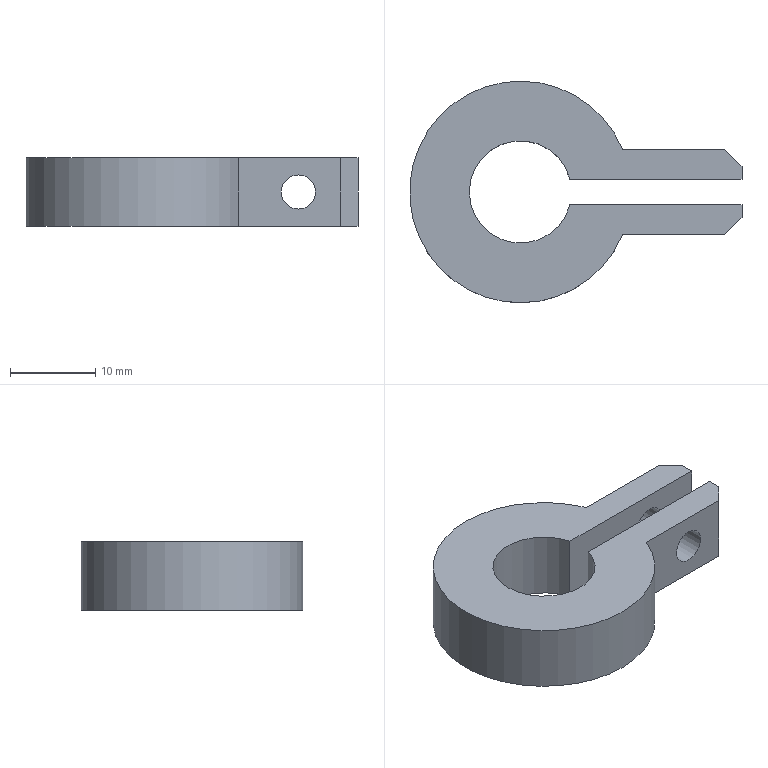Component | NX | RETAINING_RING | 1 solid | 14 faces | box 39 x 26 x 8 mm | volume 3807 mm3 | plane 10 | cylinder 4 | commonest cylinder face diameters 4.013 x2 26 x1 12 x1
STEP:
#1=CARTESIAN_POINT('',(0.,0.,0.));
#2=DIRECTION('',(0.,0.,1.));
#3=DIRECTION('',(1.,0.,0.));
#4=AXIS2_PLACEMENT_3D('',#1,#2,#3);
#5=CARTESIAN_POINT('',(33.5,3.,100.5));
#6=VERTEX_POINT('',#5);
#7=CARTESIAN_POINT('',(33.5,1.5,100.5));
#8=VERTEX_POINT('',#7);
#9=CARTESIAN_POINT('',(33.5,-0.,100.5));
#10=DIRECTION('',(0.,-1.,0.));
#11=VECTOR('',#10,1.);
#12=LINE('',#9,#11);
#13=CARTESIAN_POINT('',(33.5,-0.,108.5));
#14=DIRECTION('',(1.,0.,0.));
#15=DIRECTION('',(0.,0.,-1.));
#16=AXIS2_PLACEMENT_3D('',#13,#14,#15);
#17=PLANE('',#16);
#18=CARTESIAN_POINT('',(8.,0.));
#19=DIRECTION('',(0.,-1.));
#20=VECTOR('',#19,1.);
#21=LINE('',#18,#20);
#22=(GEOMETRIC_REPRESENTATION_CONTEXT(2)PARAMETRIC_REPRESENTATION_CONTEXT()REPRESENTATION_CONTEXT('',''));
#23=DEFINITIONAL_REPRESENTATION('',(#21),#22);
#24=PCURVE('',#17,#23);
#25=CARTESIAN_POINT('',(7.5,-0.,100.5));
#26=DIRECTION('',(0.,0.,-1.));
#27=DIRECTION('',(-1.,0.,0.));
#28=AXIS2_PLACEMENT_3D('',#25,#26,#27);
#29=PLANE('',#28);
#30=CARTESIAN_POINT('',(-26.,0.));
#31=DIRECTION('',(0.,-1.));
#32=VECTOR('',#31,1.);
#33=LINE('',#30,#32);
#34=(GEOMETRIC_REPRESENTATION_CONTEXT(2)PARAMETRIC_REPRESENTATION_CONTEXT()REPRESENTATION_CONTEXT('',''));
#35=DEFINITIONAL_REPRESENTATION('',(#33),#34);
#36=PCURVE('',#29,#35);
#37=SURFACE_CURVE('',#12,(#24,#36),.PCURVE_S1.);
#38=EDGE_CURVE('',#6,#8,#37,.T.);
#39=ORIENTED_EDGE('',*,*,#38,.F.);
#40=CARTESIAN_POINT('',(33.5,3.,108.5));
#41=VERTEX_POINT('',#40);
#42=CARTESIAN_POINT('',(33.5,3.,108.5));
#43=DIRECTION('',(0.,0.,1.));
#44=VECTOR('',#43,1.);
#45=LINE('',#42,#44);
#46=CARTESIAN_POINT('',(0.,3.));
#47=DIRECTION('',(-1.,0.));
#48=VECTOR('',#47,1.);
#49=LINE('',#46,#48);
#50=(GEOMETRIC_REPRESENTATION_CONTEXT(2)PARAMETRIC_REPRESENTATION_CONTEXT()REPRESENTATION_CONTEXT('',''));
#51=DEFINITIONAL_REPRESENTATION('',(#49),#50);
#52=PCURVE('',#17,#51);
#53=CARTESIAN_POINT('',(31.5,5.,108.5));
#54=DIRECTION('',(-0.7071,-0.7071,0.));
#55=DIRECTION('',(0.,0.,-1.));
#56=AXIS2_PLACEMENT_3D('',#53,#54,#55);
#57=PLANE('',#56);
#58=CARTESIAN_POINT('',(0.,2.828));
#59=DIRECTION('',(-1.,0.));
#60=VECTOR('',#59,1.);
#61=LINE('',#58,#60);
#62=(GEOMETRIC_REPRESENTATION_CONTEXT(2)PARAMETRIC_REPRESENTATION_CONTEXT()REPRESENTATION_CONTEXT('',''));
#63=DEFINITIONAL_REPRESENTATION('',(#61),#62);
#64=PCURVE('',#57,#63);
#65=SURFACE_CURVE('',#45,(#52,#64),.PCURVE_S1.);
#66=EDGE_CURVE('',#6,#41,#65,.T.);
#67=ORIENTED_EDGE('',*,*,#66,.T.);
#68=CARTESIAN_POINT('',(33.5,1.5,108.5));
#69=VERTEX_POINT('',#68);
#70=CARTESIAN_POINT('',(33.5,5.,108.5));
#71=DIRECTION('',(0.,-1.,0.));
#72=VECTOR('',#71,1.);
#73=LINE('',#70,#72);
#74=CARTESIAN_POINT('',(0.,5.));
#75=DIRECTION('',(0.,-1.));
#76=VECTOR('',#75,1.);
#77=LINE('',#74,#76);
#78=(GEOMETRIC_REPRESENTATION_CONTEXT(2)PARAMETRIC_REPRESENTATION_CONTEXT()REPRESENTATION_CONTEXT('',''));
#79=DEFINITIONAL_REPRESENTATION('',(#77),#78);
#80=PCURVE('',#17,#79);
#81=CARTESIAN_POINT('',(7.5,-0.,108.5));
#82=DIRECTION('',(0.,0.,-1.));
#83=DIRECTION('',(-1.,0.,0.));
#84=AXIS2_PLACEMENT_3D('',#81,#82,#83);
#85=PLANE('',#84);
#86=CARTESIAN_POINT('',(-26.,5.));
#87=DIRECTION('',(0.,-1.));
#88=VECTOR('',#87,1.);
#89=LINE('',#86,#88);
#90=(GEOMETRIC_REPRESENTATION_CONTEXT(2)PARAMETRIC_REPRESENTATION_CONTEXT()REPRESENTATION_CONTEXT('',''));
#91=DEFINITIONAL_REPRESENTATION('',(#89),#90);
#92=PCURVE('',#85,#91);
#93=SURFACE_CURVE('',#73,(#80,#92),.PCURVE_S1.);
#94=EDGE_CURVE('',#41,#69,#93,.T.);
#95=ORIENTED_EDGE('',*,*,#94,.T.);
#96=CARTESIAN_POINT('',(33.5,1.5,108.5));
#97=DIRECTION('',(0.,0.,1.));
#98=VECTOR('',#97,1.);
#99=LINE('',#96,#98);
#100=CARTESIAN_POINT('',(0.,1.5));
#101=DIRECTION('',(-1.,0.));
#102=VECTOR('',#101,1.);
#103=LINE('',#100,#102);
#104=(GEOMETRIC_REPRESENTATION_CONTEXT(2)PARAMETRIC_REPRESENTATION_CONTEXT()REPRESENTATION_CONTEXT('',''));
#105=DEFINITIONAL_REPRESENTATION('',(#103),#104);
#106=PCURVE('',#17,#105);
#107=CARTESIAN_POINT('',(36.5,1.5,95.5));
#108=DIRECTION('',(0.,1.,0.));
#109=DIRECTION('',(0.,0.,1.));
#110=AXIS2_PLACEMENT_3D('',#107,#108,#109);
#111=PLANE('',#110);
#112=CARTESIAN_POINT('',(13.,-3.));
#113=DIRECTION('',(1.,0.));
#114=VECTOR('',#113,1.);
#115=LINE('',#112,#114);
#116=(GEOMETRIC_REPRESENTATION_CONTEXT(2)PARAMETRIC_REPRESENTATION_CONTEXT()REPRESENTATION_CONTEXT('',''));
#117=DEFINITIONAL_REPRESENTATION('',(#115),#116);
#118=PCURVE('',#111,#117);
#119=SURFACE_CURVE('',#99,(#106,#118),.PCURVE_S1.);
#120=EDGE_CURVE('',#8,#69,#119,.T.);
#121=ORIENTED_EDGE('',*,*,#120,.F.);
#122=EDGE_LOOP('',(#39,#67,#95,#121));
#123=FACE_BOUND('',#122,.T.);
#124=ADVANCED_FACE('',(#123),#17,.T.);
#125=CARTESIAN_POINT('',(31.5,-5.,108.5));
#126=VERTEX_POINT('',#125);
#127=CARTESIAN_POINT('',(19.5,-5.,108.5));
#128=VERTEX_POINT('',#127);
#129=CARTESIAN_POINT('',(33.5,-5.,108.5));
#130=DIRECTION('',(-1.,0.,0.));
#131=VECTOR('',#130,1.);
#132=LINE('',#129,#131);
#133=CARTESIAN_POINT('',(-26.,-5.));
#134=DIRECTION('',(1.,0.));
#135=VECTOR('',#134,1.);
#136=LINE('',#133,#135);
#137=(GEOMETRIC_REPRESENTATION_CONTEXT(2)PARAMETRIC_REPRESENTATION_CONTEXT()REPRESENTATION_CONTEXT('',''));
#138=DEFINITIONAL_REPRESENTATION('',(#136),#137);
#139=PCURVE('',#85,#138);
#140=CARTESIAN_POINT('',(33.5,-5.,108.5));
#141=DIRECTION('',(0.,-1.,0.));
#142=DIRECTION('',(0.,0.,-1.));
#143=AXIS2_PLACEMENT_3D('',#140,#141,#142);
#144=PLANE('',#143);
#145=CARTESIAN_POINT('',(0.,0.));
#146=DIRECTION('',(0.,-1.));
#147=VECTOR('',#146,1.);
#148=LINE('',#145,#147);
#149=(GEOMETRIC_REPRESENTATION_CONTEXT(2)PARAMETRIC_REPRESENTATION_CONTEXT()REPRESENTATION_CONTEXT('',''));
#150=DEFINITIONAL_REPRESENTATION('',(#148),#149);
#151=PCURVE('',#144,#150);
#152=SURFACE_CURVE('',#132,(#139,#151),.PCURVE_S1.);
#153=EDGE_CURVE('',#126,#128,#152,.T.);
#154=ORIENTED_EDGE('',*,*,#153,.F.);
#155=CARTESIAN_POINT('',(33.5,-3.,108.5));
#156=VERTEX_POINT('',#155);
#157=CARTESIAN_POINT('',(33.5,-3.,108.5));
#158=DIRECTION('',(0.7071,0.7071,0.));
#159=VECTOR('',#158,1.);
#160=LINE('',#157,#159);
#161=CARTESIAN_POINT('',(-26.,-3.));
#162=DIRECTION('',(-0.7071,0.7071));
#163=VECTOR('',#162,1.);
#164=LINE('',#161,#163);
#165=(GEOMETRIC_REPRESENTATION_CONTEXT(2)PARAMETRIC_REPRESENTATION_CONTEXT()REPRESENTATION_CONTEXT('',''));
#166=DEFINITIONAL_REPRESENTATION('',(#164),#165);
#167=PCURVE('',#85,#166);
#168=CARTESIAN_POINT('',(33.5,-3.,108.5));
#169=DIRECTION('',(-0.7071,0.7071,0.));
#170=DIRECTION('',(0.,0.,-1.));
#171=AXIS2_PLACEMENT_3D('',#168,#169,#170);
#172=PLANE('',#171);
#173=CARTESIAN_POINT('',(0.,0.));
#174=DIRECTION('',(0.,-1.));
#175=VECTOR('',#174,1.);
#176=LINE('',#173,#175);
#177=(GEOMETRIC_REPRESENTATION_CONTEXT(2)PARAMETRIC_REPRESENTATION_CONTEXT()REPRESENTATION_CONTEXT('',''));
#178=DEFINITIONAL_REPRESENTATION('',(#176),#177);
#179=PCURVE('',#172,#178);
#180=SURFACE_CURVE('',#160,(#167,#179),.PCURVE_S1.);
#181=EDGE_CURVE('',#126,#156,#180,.T.);
#182=ORIENTED_EDGE('',*,*,#181,.T.);
#183=CARTESIAN_POINT('',(33.5,-1.5,108.5));
#184=VERTEX_POINT('',#183);
#185=CARTESIAN_POINT('',(33.5,5.,108.5));
#186=DIRECTION('',(0.,-1.,0.));
#187=VECTOR('',#186,1.);
#188=LINE('',#185,#187);
#189=CARTESIAN_POINT('',(-26.,5.));
#190=DIRECTION('',(0.,-1.));
#191=VECTOR('',#190,1.);
#192=LINE('',#189,#191);
#193=(GEOMETRIC_REPRESENTATION_CONTEXT(2)PARAMETRIC_REPRESENTATION_CONTEXT()REPRESENTATION_CONTEXT('',''));
#194=DEFINITIONAL_REPRESENTATION('',(#192),#193);
#195=PCURVE('',#85,#194);
#196=CARTESIAN_POINT('',(33.5,-0.,108.5));
#197=DIRECTION('',(1.,0.,0.));
#198=DIRECTION('',(0.,0.,-1.));
#199=AXIS2_PLACEMENT_3D('',#196,#197,#198);
#200=PLANE('',#199);
#201=CARTESIAN_POINT('',(0.,5.));
#202=DIRECTION('',(0.,-1.));
#203=VECTOR('',#202,1.);
#204=LINE('',#201,#203);
#205=(GEOMETRIC_REPRESENTATION_CONTEXT(2)PARAMETRIC_REPRESENTATION_CONTEXT()REPRESENTATION_CONTEXT('',''));
#206=DEFINITIONAL_REPRESENTATION('',(#204),#205);
#207=PCURVE('',#200,#206);
#208=SURFACE_CURVE('',#188,(#195,#207),.PCURVE_S1.);
#209=EDGE_CURVE('',#184,#156,#208,.T.);
#210=ORIENTED_EDGE('',*,*,#209,.F.);
#211=CARTESIAN_POINT('',(13.309,-1.5,108.5));
#212=VERTEX_POINT('',#211);
#213=CARTESIAN_POINT('',(12.,-1.5,108.5));
#214=DIRECTION('',(1.,0.,0.));
#215=VECTOR('',#214,1.);
#216=LINE('',#213,#215);
#217=CARTESIAN_POINT('',(-4.5,-1.5));
#218=DIRECTION('',(-1.,0.));
#219=VECTOR('',#218,1.);
#220=LINE('',#217,#219);
#221=(GEOMETRIC_REPRESENTATION_CONTEXT(2)PARAMETRIC_REPRESENTATION_CONTEXT()REPRESENTATION_CONTEXT('',''));
#222=DEFINITIONAL_REPRESENTATION('',(#220),#221);
#223=PCURVE('',#85,#222);
#224=CARTESIAN_POINT('',(12.,-1.5,95.5));
#225=DIRECTION('',(0.,-1.,0.));
#226=DIRECTION('',(0.,0.,-1.));
#227=AXIS2_PLACEMENT_3D('',#224,#225,#226);
#228=PLANE('',#227);
#229=CARTESIAN_POINT('',(-13.,0.));
#230=DIRECTION('',(0.,1.));
#231=VECTOR('',#230,1.);
#232=LINE('',#229,#231);
#233=(GEOMETRIC_REPRESENTATION_CONTEXT(2)PARAMETRIC_REPRESENTATION_CONTEXT()REPRESENTATION_CONTEXT('',''));
#234=DEFINITIONAL_REPRESENTATION('',(#232),#233);
#235=PCURVE('',#228,#234);
#236=SURFACE_CURVE('',#216,(#223,#235),.PCURVE_S1.);
#237=EDGE_CURVE('',#212,#184,#236,.T.);
#238=ORIENTED_EDGE('',*,*,#237,.F.);
#239=CARTESIAN_POINT('',(13.309,1.5,108.5));
#240=VERTEX_POINT('',#239);
#241=CARTESIAN_POINT('',(7.5,-0.,108.5));
#242=DIRECTION('',(0.,0.,-1.));
#243=DIRECTION('',(1.,0.,0.));
#244=AXIS2_PLACEMENT_3D('',#241,#242,#243);
#245=CIRCLE('',#244,6.);
#246=CARTESIAN_POINT('',(0.,0.));
#247=DIRECTION('',(-1.,0.));
#248=AXIS2_PLACEMENT_2D('',#246,#247);
#249=CIRCLE('',#248,6.);
#250=(GEOMETRIC_REPRESENTATION_CONTEXT(2)PARAMETRIC_REPRESENTATION_CONTEXT()REPRESENTATION_CONTEXT('',''));
#251=DEFINITIONAL_REPRESENTATION('',(#249),#250);
#252=PCURVE('',#85,#251);
#253=CARTESIAN_POINT('',(7.5,-0.,108.5));
#254=DIRECTION('',(0.,0.,-1.));
#255=DIRECTION('',(-1.,0.,0.));
#256=AXIS2_PLACEMENT_3D('',#253,#254,#255);
#257=CYLINDRICAL_SURFACE('',#256,6.);
#258=CARTESIAN_POINT('',(3.142,0.));
#259=DIRECTION('',(1.,0.));
#260=VECTOR('',#259,1.);
#261=LINE('',#258,#260);
#262=(GEOMETRIC_REPRESENTATION_CONTEXT(2)PARAMETRIC_REPRESENTATION_CONTEXT()REPRESENTATION_CONTEXT('',''));
#263=DEFINITIONAL_REPRESENTATION('',(#261),#262);
#264=PCURVE('',#257,#263);
#265=SURFACE_CURVE('',#245,(#252,#264),.PCURVE_S1.);
#266=EDGE_CURVE('',#212,#240,#265,.T.);
#267=ORIENTED_EDGE('',*,*,#266,.T.);
#268=CARTESIAN_POINT('',(36.5,1.5,108.5));
#269=DIRECTION('',(-1.,0.,0.));
#270=VECTOR('',#269,1.);
#271=LINE('',#268,#270);
#272=CARTESIAN_POINT('',(-29.,1.5));
#273=DIRECTION('',(1.,0.));
#274=VECTOR('',#273,1.);
#275=LINE('',#272,#274);
#276=(GEOMETRIC_REPRESENTATION_CONTEXT(2)PARAMETRIC_REPRESENTATION_CONTEXT()REPRESENTATION_CONTEXT('',''));
#277=DEFINITIONAL_REPRESENTATION('',(#275),#276);
#278=PCURVE('',#85,#277);
#279=CARTESIAN_POINT('',(13.,0.));
#280=DIRECTION('',(0.,-1.));
#281=VECTOR('',#280,1.);
#282=LINE('',#279,#281);
#283=(GEOMETRIC_REPRESENTATION_CONTEXT(2)PARAMETRIC_REPRESENTATION_CONTEXT()REPRESENTATION_CONTEXT('',''));
#284=DEFINITIONAL_REPRESENTATION('',(#282),#283);
#285=PCURVE('',#111,#284);
#286=SURFACE_CURVE('',#271,(#278,#285),.PCURVE_S1.);
#287=EDGE_CURVE('',#69,#240,#286,.T.);
#288=ORIENTED_EDGE('',*,*,#287,.F.);
#289=ORIENTED_EDGE('',*,*,#94,.F.);
#290=CARTESIAN_POINT('',(31.5,5.,108.5));
#291=VERTEX_POINT('',#290);
#292=CARTESIAN_POINT('',(31.5,5.,108.5));
#293=DIRECTION('',(-0.7071,0.7071,0.));
#294=VECTOR('',#293,1.);
#295=LINE('',#292,#294);
#296=CARTESIAN_POINT('',(-24.,5.));
#297=DIRECTION('',(0.7071,0.7071));
#298=VECTOR('',#297,1.);
#299=LINE('',#296,#298);
#300=(GEOMETRIC_REPRESENTATION_CONTEXT(2)PARAMETRIC_REPRESENTATION_CONTEXT()REPRESENTATION_CONTEXT('',''));
#301=DEFINITIONAL_REPRESENTATION('',(#299),#300);
#302=PCURVE('',#85,#301);
#303=CARTESIAN_POINT('',(0.,0.));
#304=DIRECTION('',(0.,-1.));
#305=VECTOR('',#304,1.);
#306=LINE('',#303,#305);
#307=(GEOMETRIC_REPRESENTATION_CONTEXT(2)PARAMETRIC_REPRESENTATION_CONTEXT()REPRESENTATION_CONTEXT('',''));
#308=DEFINITIONAL_REPRESENTATION('',(#306),#307);
#309=PCURVE('',#57,#308);
#310=SURFACE_CURVE('',#295,(#302,#309),.PCURVE_S1.);
#311=EDGE_CURVE('',#41,#291,#310,.T.);
#312=ORIENTED_EDGE('',*,*,#311,.T.);
#313=CARTESIAN_POINT('',(19.5,5.,108.5));
#314=VERTEX_POINT('',#313);
#315=CARTESIAN_POINT('',(19.5,5.,108.5));
#316=DIRECTION('',(1.,0.,0.));
#317=VECTOR('',#316,1.);
#318=LINE('',#315,#317);
#319=CARTESIAN_POINT('',(-12.,5.));
#320=DIRECTION('',(-1.,0.));
#321=VECTOR('',#320,1.);
#322=LINE('',#319,#321);
#323=(GEOMETRIC_REPRESENTATION_CONTEXT(2)PARAMETRIC_REPRESENTATION_CONTEXT()REPRESENTATION_CONTEXT('',''));
#324=DEFINITIONAL_REPRESENTATION('',(#322),#323);
#325=PCURVE('',#85,#324);
#326=CARTESIAN_POINT('',(19.5,5.,108.5));
#327=DIRECTION('',(0.,1.,0.));
#328=DIRECTION('',(0.,0.,1.));
#329=AXIS2_PLACEMENT_3D('',#326,#327,#328);
#330=PLANE('',#329);
#331=CARTESIAN_POINT('',(0.,0.));
#332=DIRECTION('',(0.,1.));
#333=VECTOR('',#332,1.);
#334=LINE('',#331,#333);
#335=(GEOMETRIC_REPRESENTATION_CONTEXT(2)PARAMETRIC_REPRESENTATION_CONTEXT()REPRESENTATION_CONTEXT('',''));
#336=DEFINITIONAL_REPRESENTATION('',(#334),#335);
#337=PCURVE('',#330,#336);
#338=SURFACE_CURVE('',#318,(#325,#337),.PCURVE_S1.);
#339=EDGE_CURVE('',#314,#291,#338,.T.);
#340=ORIENTED_EDGE('',*,*,#339,.F.);
#341=CARTESIAN_POINT('',(7.5,-0.,108.5));
#342=DIRECTION('',(0.,0.,-1.));
#343=DIRECTION('',(1.,0.,0.));
#344=AXIS2_PLACEMENT_3D('',#341,#342,#343);
#345=CIRCLE('',#344,13.);
#346=CARTESIAN_POINT('',(0.,0.));
#347=DIRECTION('',(-1.,0.));
#348=AXIS2_PLACEMENT_2D('',#346,#347);
#349=CIRCLE('',#348,13.);
#350=(GEOMETRIC_REPRESENTATION_CONTEXT(2)PARAMETRIC_REPRESENTATION_CONTEXT()REPRESENTATION_CONTEXT('',''));
#351=DEFINITIONAL_REPRESENTATION('',(#349),#350);
#352=PCURVE('',#85,#351);
#353=CARTESIAN_POINT('',(7.5,-0.,108.5));
#354=DIRECTION('',(0.,0.,-1.));
#355=DIRECTION('',(-1.,0.,0.));
#356=AXIS2_PLACEMENT_3D('',#353,#354,#355);
#357=CYLINDRICAL_SURFACE('',#356,13.);
#358=CARTESIAN_POINT('',(3.142,0.));
#359=DIRECTION('',(1.,0.));
#360=VECTOR('',#359,1.);
#361=LINE('',#358,#360);
#362=(GEOMETRIC_REPRESENTATION_CONTEXT(2)PARAMETRIC_REPRESENTATION_CONTEXT()REPRESENTATION_CONTEXT('',''));
#363=DEFINITIONAL_REPRESENTATION('',(#361),#362);
#364=PCURVE('',#357,#363);
#365=SURFACE_CURVE('',#345,(#352,#364),.PCURVE_S1.);
#366=EDGE_CURVE('',#128,#314,#365,.T.);
#367=ORIENTED_EDGE('',*,*,#366,.F.);
#368=EDGE_LOOP('',(#154,#182,#210,#238,#267,#288,#289,#312,#340,#367));
#369=FACE_BOUND('',#368,.T.);
#370=ADVANCED_FACE('',(#369),#85,.F.);
#371=CARTESIAN_POINT('',(19.5,-5.,100.5));
#372=VERTEX_POINT('',#371);
#373=CARTESIAN_POINT('',(19.5,5.,100.5));
#374=VERTEX_POINT('',#373);
#375=CARTESIAN_POINT('',(7.5,-0.,100.5));
#376=DIRECTION('',(0.,0.,-1.));
#377=DIRECTION('',(1.,0.,0.));
#378=AXIS2_PLACEMENT_3D('',#375,#376,#377);
#379=CIRCLE('',#378,13.);
#380=CARTESIAN_POINT('',(3.142,8.));
#381=DIRECTION('',(1.,0.));
#382=VECTOR('',#381,1.);
#383=LINE('',#380,#382);
#384=(GEOMETRIC_REPRESENTATION_CONTEXT(2)PARAMETRIC_REPRESENTATION_CONTEXT()REPRESENTATION_CONTEXT('',''));
#385=DEFINITIONAL_REPRESENTATION('',(#383),#384);
#386=PCURVE('',#357,#385);
#387=CARTESIAN_POINT('',(0.,0.));
#388=DIRECTION('',(-1.,0.));
#389=AXIS2_PLACEMENT_2D('',#387,#388);
#390=CIRCLE('',#389,13.);
#391=(GEOMETRIC_REPRESENTATION_CONTEXT(2)PARAMETRIC_REPRESENTATION_CONTEXT()REPRESENTATION_CONTEXT('',''));
#392=DEFINITIONAL_REPRESENTATION('',(#390),#391);
#393=PCURVE('',#29,#392);
#394=SURFACE_CURVE('',#379,(#386,#393),.PCURVE_S1.);
#395=EDGE_CURVE('',#372,#374,#394,.T.);
#396=ORIENTED_EDGE('',*,*,#395,.F.);
#397=CARTESIAN_POINT('',(19.5,-5.,108.5));
#398=DIRECTION('',(0.,0.,-1.));
#399=VECTOR('',#398,1.);
#400=LINE('',#397,#399);
#401=CARTESIAN_POINT('',(3.536,0.));
#402=DIRECTION('',(0.,1.));
#403=VECTOR('',#402,1.);
#404=LINE('',#401,#403);
#405=(GEOMETRIC_REPRESENTATION_CONTEXT(2)PARAMETRIC_REPRESENTATION_CONTEXT()REPRESENTATION_CONTEXT('',''));
#406=DEFINITIONAL_REPRESENTATION('',(#404),#405);
#407=PCURVE('',#357,#406);
#408=CARTESIAN_POINT('',(0.,-14.));
#409=DIRECTION('',(1.,0.));
#410=VECTOR('',#409,1.);
#411=LINE('',#408,#410);
#412=(GEOMETRIC_REPRESENTATION_CONTEXT(2)PARAMETRIC_REPRESENTATION_CONTEXT()REPRESENTATION_CONTEXT('',''));
#413=DEFINITIONAL_REPRESENTATION('',(#411),#412);
#414=PCURVE('',#144,#413);
#415=SURFACE_CURVE('',#400,(#407,#414),.PCURVE_S1.);
#416=EDGE_CURVE('',#128,#372,#415,.T.);
#417=ORIENTED_EDGE('',*,*,#416,.F.);
#418=ORIENTED_EDGE('',*,*,#366,.T.);
#419=CARTESIAN_POINT('',(19.5,5.,108.5));
#420=DIRECTION('',(0.,0.,-1.));
#421=VECTOR('',#420,1.);
#422=LINE('',#419,#421);
#423=CARTESIAN_POINT('',(9.03,0.));
#424=DIRECTION('',(0.,1.));
#425=VECTOR('',#424,1.);
#426=LINE('',#423,#425);
#427=(GEOMETRIC_REPRESENTATION_CONTEXT(2)PARAMETRIC_REPRESENTATION_CONTEXT()REPRESENTATION_CONTEXT('',''));
#428=DEFINITIONAL_REPRESENTATION('',(#426),#427);
#429=PCURVE('',#357,#428);
#430=CARTESIAN_POINT('',(0.,0.));
#431=DIRECTION('',(-1.,0.));
#432=VECTOR('',#431,1.);
#433=LINE('',#430,#432);
#434=(GEOMETRIC_REPRESENTATION_CONTEXT(2)PARAMETRIC_REPRESENTATION_CONTEXT()REPRESENTATION_CONTEXT('',''));
#435=DEFINITIONAL_REPRESENTATION('',(#433),#434);
#436=PCURVE('',#330,#435);
#437=SURFACE_CURVE('',#422,(#429,#436),.PCURVE_S1.);
#438=EDGE_CURVE('',#314,#374,#437,.T.);
#439=ORIENTED_EDGE('',*,*,#438,.T.);
#440=EDGE_LOOP('',(#396,#417,#418,#439));
#441=FACE_BOUND('',#440,.T.);
#442=ADVANCED_FACE('',(#441),#357,.T.);
#443=CARTESIAN_POINT('',(26.5,5.,106.507));
#444=VERTEX_POINT('',#443);
#445=CARTESIAN_POINT('',(26.5,5.,104.5));
#446=DIRECTION('',(0.,1.,0.));
#447=DIRECTION('',(0.,0.,1.));
#448=AXIS2_PLACEMENT_3D('',#445,#446,#447);
#449=CIRCLE('',#448,2.007);
#450=CARTESIAN_POINT('',(-4.,7.));
#451=DIRECTION('',(1.,0.));
#452=AXIS2_PLACEMENT_2D('',#450,#451);
#453=CIRCLE('',#452,2.007);
#454=(GEOMETRIC_REPRESENTATION_CONTEXT(2)PARAMETRIC_REPRESENTATION_CONTEXT()REPRESENTATION_CONTEXT('',''));
#455=DEFINITIONAL_REPRESENTATION('',(#453),#454);
#456=PCURVE('',#330,#455);
#457=CARTESIAN_POINT('',(26.5,-6.,104.5));
#458=DIRECTION('',(0.,1.,0.));
#459=DIRECTION('',(1.,0.,0.));
#460=AXIS2_PLACEMENT_3D('',#457,#458,#459);
#461=CYLINDRICAL_SURFACE('',#460,2.007);
#462=CARTESIAN_POINT('',(4.712,11.));
#463=DIRECTION('',(1.,0.));
#464=VECTOR('',#463,1.);
#465=LINE('',#462,#464);
#466=(GEOMETRIC_REPRESENTATION_CONTEXT(2)PARAMETRIC_REPRESENTATION_CONTEXT()REPRESENTATION_CONTEXT('',''));
#467=DEFINITIONAL_REPRESENTATION('',(#465),#466);
#468=PCURVE('',#461,#467);
#469=SURFACE_CURVE('',#449,(#456,#468),.PCURVE_S1.);
#470=EDGE_CURVE('',#444,#444,#469,.T.);
#471=ORIENTED_EDGE('',*,*,#470,.F.);
#472=EDGE_LOOP('',(#471));
#473=FACE_BOUND('',#472,.T.);
#474=ORIENTED_EDGE('',*,*,#339,.T.);
#475=CARTESIAN_POINT('',(31.5,5.,100.5));
#476=VERTEX_POINT('',#475);
#477=CARTESIAN_POINT('',(31.5,5.,108.5));
#478=DIRECTION('',(0.,0.,-1.));
#479=VECTOR('',#478,1.);
#480=LINE('',#477,#479);
#481=CARTESIAN_POINT('',(0.,12.));
#482=DIRECTION('',(-1.,0.));
#483=VECTOR('',#482,1.);
#484=LINE('',#481,#483);
#485=(GEOMETRIC_REPRESENTATION_CONTEXT(2)PARAMETRIC_REPRESENTATION_CONTEXT()REPRESENTATION_CONTEXT('',''));
#486=DEFINITIONAL_REPRESENTATION('',(#484),#485);
#487=PCURVE('',#330,#486);
#488=CARTESIAN_POINT('',(0.,0.));
#489=DIRECTION('',(1.,0.));
#490=VECTOR('',#489,1.);
#491=LINE('',#488,#490);
#492=(GEOMETRIC_REPRESENTATION_CONTEXT(2)PARAMETRIC_REPRESENTATION_CONTEXT()REPRESENTATION_CONTEXT('',''));
#493=DEFINITIONAL_REPRESENTATION('',(#491),#492);
#494=PCURVE('',#57,#493);
#495=SURFACE_CURVE('',#480,(#487,#494),.PCURVE_S1.);
#496=EDGE_CURVE('',#291,#476,#495,.T.);
#497=ORIENTED_EDGE('',*,*,#496,.T.);
#498=CARTESIAN_POINT('',(19.5,5.,100.5));
#499=DIRECTION('',(1.,0.,0.));
#500=VECTOR('',#499,1.);
#501=LINE('',#498,#500);
#502=CARTESIAN_POINT('',(-8.,0.));
#503=DIRECTION('',(0.,1.));
#504=VECTOR('',#503,1.);
#505=LINE('',#502,#504);
#506=(GEOMETRIC_REPRESENTATION_CONTEXT(2)PARAMETRIC_REPRESENTATION_CONTEXT()REPRESENTATION_CONTEXT('',''));
#507=DEFINITIONAL_REPRESENTATION('',(#505),#506);
#508=PCURVE('',#330,#507);
#509=CARTESIAN_POINT('',(-12.,5.));
#510=DIRECTION('',(-1.,0.));
#511=VECTOR('',#510,1.);
#512=LINE('',#509,#511);
#513=(GEOMETRIC_REPRESENTATION_CONTEXT(2)PARAMETRIC_REPRESENTATION_CONTEXT()REPRESENTATION_CONTEXT('',''));
#514=DEFINITIONAL_REPRESENTATION('',(#512),#513);
#515=PCURVE('',#29,#514);
#516=SURFACE_CURVE('',#501,(#508,#515),.PCURVE_S1.);
#517=EDGE_CURVE('',#374,#476,#516,.T.);
#518=ORIENTED_EDGE('',*,*,#517,.F.);
#519=ORIENTED_EDGE('',*,*,#438,.F.);
#520=EDGE_LOOP('',(#474,#497,#518,#519));
#521=FACE_BOUND('',#520,.T.);
#522=ADVANCED_FACE('',(#473,#521),#330,.T.);
#523=ORIENTED_EDGE('',*,*,#209,.T.);
#524=CARTESIAN_POINT('',(33.5,-3.,100.5));
#525=VERTEX_POINT('',#524);
#526=CARTESIAN_POINT('',(33.5,-3.,108.5));
#527=DIRECTION('',(0.,0.,-1.));
#528=VECTOR('',#527,1.);
#529=LINE('',#526,#528);
#530=CARTESIAN_POINT('',(0.,-3.));
#531=DIRECTION('',(1.,0.));
#532=VECTOR('',#531,1.);
#533=LINE('',#530,#532);
#534=(GEOMETRIC_REPRESENTATION_CONTEXT(2)PARAMETRIC_REPRESENTATION_CONTEXT()REPRESENTATION_CONTEXT('',''));
#535=DEFINITIONAL_REPRESENTATION('',(#533),#534);
#536=PCURVE('',#200,#535);
#537=CARTESIAN_POINT('',(0.,0.));
#538=DIRECTION('',(1.,0.));
#539=VECTOR('',#538,1.);
#540=LINE('',#537,#539);
#541=(GEOMETRIC_REPRESENTATION_CONTEXT(2)PARAMETRIC_REPRESENTATION_CONTEXT()REPRESENTATION_CONTEXT('',''));
#542=DEFINITIONAL_REPRESENTATION('',(#540),#541);
#543=PCURVE('',#172,#542);
#544=SURFACE_CURVE('',#529,(#536,#543),.PCURVE_S1.);
#545=EDGE_CURVE('',#156,#525,#544,.T.);
#546=ORIENTED_EDGE('',*,*,#545,.T.);
#547=CARTESIAN_POINT('',(33.5,-1.5,100.5));
#548=VERTEX_POINT('',#547);
#549=CARTESIAN_POINT('',(33.5,-0.,100.5));
#550=DIRECTION('',(0.,-1.,0.));
#551=VECTOR('',#550,1.);
#552=LINE('',#549,#551);
#553=CARTESIAN_POINT('',(8.,0.));
#554=DIRECTION('',(0.,-1.));
#555=VECTOR('',#554,1.);
#556=LINE('',#553,#555);
#557=(GEOMETRIC_REPRESENTATION_CONTEXT(2)PARAMETRIC_REPRESENTATION_CONTEXT()REPRESENTATION_CONTEXT('',''));
#558=DEFINITIONAL_REPRESENTATION('',(#556),#557);
#559=PCURVE('',#200,#558);
#560=CARTESIAN_POINT('',(-26.,0.));
#561=DIRECTION('',(0.,-1.));
#562=VECTOR('',#561,1.);
#563=LINE('',#560,#562);
#564=(GEOMETRIC_REPRESENTATION_CONTEXT(2)PARAMETRIC_REPRESENTATION_CONTEXT()REPRESENTATION_CONTEXT('',''));
#565=DEFINITIONAL_REPRESENTATION('',(#563),#564);
#566=PCURVE('',#29,#565);
#567=SURFACE_CURVE('',#552,(#559,#566),.PCURVE_S1.);
#568=EDGE_CURVE('',#548,#525,#567,.T.);
#569=ORIENTED_EDGE('',*,*,#568,.F.);
#570=CARTESIAN_POINT('',(33.5,-1.5,108.5));
#571=DIRECTION('',(0.,0.,-1.));
#572=VECTOR('',#571,1.);
#573=LINE('',#570,#572);
#574=CARTESIAN_POINT('',(0.,-1.5));
#575=DIRECTION('',(1.,0.));
#576=VECTOR('',#575,1.);
#577=LINE('',#574,#576);
#578=(GEOMETRIC_REPRESENTATION_CONTEXT(2)PARAMETRIC_REPRESENTATION_CONTEXT()REPRESENTATION_CONTEXT('',''));
#579=DEFINITIONAL_REPRESENTATION('',(#577),#578);
#580=PCURVE('',#200,#579);
#581=CARTESIAN_POINT('',(-13.,21.5));
#582=DIRECTION('',(1.,0.));
#583=VECTOR('',#582,1.);
#584=LINE('',#581,#583);
#585=(GEOMETRIC_REPRESENTATION_CONTEXT(2)PARAMETRIC_REPRESENTATION_CONTEXT()REPRESENTATION_CONTEXT('',''));
#586=DEFINITIONAL_REPRESENTATION('',(#584),#585);
#587=PCURVE('',#228,#586);
#588=SURFACE_CURVE('',#573,(#580,#587),.PCURVE_S1.);
#589=EDGE_CURVE('',#184,#548,#588,.T.);
#590=ORIENTED_EDGE('',*,*,#589,.F.);
#591=EDGE_LOOP('',(#523,#546,#569,#590));
#592=FACE_BOUND('',#591,.T.);
#593=ADVANCED_FACE('',(#592),#200,.T.);
#594=CARTESIAN_POINT('',(26.5,-5.,102.493));
#595=VERTEX_POINT('',#594);
#596=CARTESIAN_POINT('',(26.5,-5.,104.5));
#597=DIRECTION('',(0.,-1.,0.));
#598=DIRECTION('',(0.,0.,-1.));
#599=AXIS2_PLACEMENT_3D('',#596,#597,#598);
#600=CIRCLE('',#599,2.007);
#601=CARTESIAN_POINT('',(4.,-7.));
#602=DIRECTION('',(1.,0.));
#603=AXIS2_PLACEMENT_2D('',#601,#602);
#604=CIRCLE('',#603,2.007);
#605=(GEOMETRIC_REPRESENTATION_CONTEXT(2)PARAMETRIC_REPRESENTATION_CONTEXT()REPRESENTATION_CONTEXT('',''));
#606=DEFINITIONAL_REPRESENTATION('',(#604),#605);
#607=PCURVE('',#144,#606);
#608=CARTESIAN_POINT('',(26.5,-6.,104.5));
#609=DIRECTION('',(0.,1.,0.));
#610=DIRECTION('',(1.,0.,0.));
#611=AXIS2_PLACEMENT_3D('',#608,#609,#610);
#612=CYLINDRICAL_SURFACE('',#611,2.007);
#613=CARTESIAN_POINT('',(7.854,1.));
#614=DIRECTION('',(-1.,0.));
#615=VECTOR('',#614,1.);
#616=LINE('',#613,#615);
#617=(GEOMETRIC_REPRESENTATION_CONTEXT(2)PARAMETRIC_REPRESENTATION_CONTEXT()REPRESENTATION_CONTEXT('',''));
#618=DEFINITIONAL_REPRESENTATION('',(#616),#617);
#619=PCURVE('',#612,#618);
#620=SURFACE_CURVE('',#600,(#607,#619),.PCURVE_S1.);
#621=EDGE_CURVE('',#595,#595,#620,.T.);
#622=ORIENTED_EDGE('',*,*,#621,.F.);
#623=EDGE_LOOP('',(#622));
#624=FACE_BOUND('',#623,.T.);
#625=CARTESIAN_POINT('',(31.5,-5.,100.5));
#626=VERTEX_POINT('',#625);
#627=CARTESIAN_POINT('',(33.5,-5.,100.5));
#628=DIRECTION('',(-1.,0.,0.));
#629=VECTOR('',#628,1.);
#630=LINE('',#627,#629);
#631=CARTESIAN_POINT('',(8.,0.));
#632=DIRECTION('',(0.,-1.));
#633=VECTOR('',#632,1.);
#634=LINE('',#631,#633);
#635=(GEOMETRIC_REPRESENTATION_CONTEXT(2)PARAMETRIC_REPRESENTATION_CONTEXT()REPRESENTATION_CONTEXT('',''));
#636=DEFINITIONAL_REPRESENTATION('',(#634),#635);
#637=PCURVE('',#144,#636);
#638=CARTESIAN_POINT('',(-26.,-5.));
#639=DIRECTION('',(1.,0.));
#640=VECTOR('',#639,1.);
#641=LINE('',#638,#640);
#642=(GEOMETRIC_REPRESENTATION_CONTEXT(2)PARAMETRIC_REPRESENTATION_CONTEXT()REPRESENTATION_CONTEXT('',''));
#643=DEFINITIONAL_REPRESENTATION('',(#641),#642);
#644=PCURVE('',#29,#643);
#645=SURFACE_CURVE('',#630,(#637,#644),.PCURVE_S1.);
#646=EDGE_CURVE('',#626,#372,#645,.T.);
#647=ORIENTED_EDGE('',*,*,#646,.F.);
#648=CARTESIAN_POINT('',(31.5,-5.,108.5));
#649=DIRECTION('',(0.,0.,1.));
#650=VECTOR('',#649,1.);
#651=LINE('',#648,#650);
#652=CARTESIAN_POINT('',(0.,-2.));
#653=DIRECTION('',(-1.,0.));
#654=VECTOR('',#653,1.);
#655=LINE('',#652,#654);
#656=(GEOMETRIC_REPRESENTATION_CONTEXT(2)PARAMETRIC_REPRESENTATION_CONTEXT()REPRESENTATION_CONTEXT('',''));
#657=DEFINITIONAL_REPRESENTATION('',(#655),#656);
#658=PCURVE('',#144,#657);
#659=CARTESIAN_POINT('',(0.,2.828));
#660=DIRECTION('',(-1.,0.));
#661=VECTOR('',#660,1.);
#662=LINE('',#659,#661);
#663=(GEOMETRIC_REPRESENTATION_CONTEXT(2)PARAMETRIC_REPRESENTATION_CONTEXT()REPRESENTATION_CONTEXT('',''));
#664=DEFINITIONAL_REPRESENTATION('',(#662),#663);
#665=PCURVE('',#172,#664);
#666=SURFACE_CURVE('',#651,(#658,#665),.PCURVE_S1.);
#667=EDGE_CURVE('',#626,#126,#666,.T.);
#668=ORIENTED_EDGE('',*,*,#667,.T.);
#669=ORIENTED_EDGE('',*,*,#153,.T.);
#670=ORIENTED_EDGE('',*,*,#416,.T.);
#671=EDGE_LOOP('',(#647,#668,#669,#670));
#672=FACE_BOUND('',#671,.T.);
#673=ADVANCED_FACE('',(#624,#672),#144,.T.);
#674=CARTESIAN_POINT('',(13.309,-1.5,100.5));
#675=VERTEX_POINT('',#674);
#676=CARTESIAN_POINT('',(13.309,-1.5,108.5));
#677=DIRECTION('',(0.,0.,-1.));
#678=VECTOR('',#677,1.);
#679=LINE('',#676,#678);
#680=CARTESIAN_POINT('',(3.394,0.));
#681=DIRECTION('',(0.,1.));
#682=VECTOR('',#681,1.);
#683=LINE('',#680,#682);
#684=(GEOMETRIC_REPRESENTATION_CONTEXT(2)PARAMETRIC_REPRESENTATION_CONTEXT()REPRESENTATION_CONTEXT('',''));
#685=DEFINITIONAL_REPRESENTATION('',(#683),#684);
#686=PCURVE('',#257,#685);
#687=CARTESIAN_POINT('',(-13.,1.309));
#688=DIRECTION('',(1.,0.));
#689=VECTOR('',#688,1.);
#690=LINE('',#687,#689);
#691=(GEOMETRIC_REPRESENTATION_CONTEXT(2)PARAMETRIC_REPRESENTATION_CONTEXT()REPRESENTATION_CONTEXT('',''));
#692=DEFINITIONAL_REPRESENTATION('',(#690),#691);
#693=PCURVE('',#228,#692);
#694=SURFACE_CURVE('',#679,(#686,#693),.PCURVE_S1.);
#695=EDGE_CURVE('',#212,#675,#694,.T.);
#696=ORIENTED_EDGE('',*,*,#695,.F.);
#697=ORIENTED_EDGE('',*,*,#266,.T.);
#698=CARTESIAN_POINT('',(13.309,1.5,100.5));
#699=VERTEX_POINT('',#698);
#700=CARTESIAN_POINT('',(13.309,1.5,108.5));
#701=DIRECTION('',(0.,0.,1.));
#702=VECTOR('',#701,1.);
#703=LINE('',#700,#702);
#704=CARTESIAN_POINT('',(9.172,0.));
#705=DIRECTION('',(0.,-1.));
#706=VECTOR('',#705,1.);
#707=LINE('',#704,#706);
#708=(GEOMETRIC_REPRESENTATION_CONTEXT(2)PARAMETRIC_REPRESENTATION_CONTEXT()REPRESENTATION_CONTEXT('',''));
#709=DEFINITIONAL_REPRESENTATION('',(#707),#708);
#710=PCURVE('',#257,#709);
#711=CARTESIAN_POINT('',(13.,-23.191));
#712=DIRECTION('',(1.,0.));
#713=VECTOR('',#712,1.);
#714=LINE('',#711,#713);
#715=(GEOMETRIC_REPRESENTATION_CONTEXT(2)PARAMETRIC_REPRESENTATION_CONTEXT()REPRESENTATION_CONTEXT('',''));
#716=DEFINITIONAL_REPRESENTATION('',(#714),#715);
#717=PCURVE('',#111,#716);
#718=SURFACE_CURVE('',#703,(#710,#717),.PCURVE_S1.);
#719=EDGE_CURVE('',#699,#240,#718,.T.);
#720=ORIENTED_EDGE('',*,*,#719,.F.);
#721=CARTESIAN_POINT('',(7.5,-0.,100.5));
#722=DIRECTION('',(0.,0.,-1.));
#723=DIRECTION('',(1.,0.,0.));
#724=AXIS2_PLACEMENT_3D('',#721,#722,#723);
#725=CIRCLE('',#724,6.);
#726=CARTESIAN_POINT('',(3.142,8.));
#727=DIRECTION('',(1.,0.));
#728=VECTOR('',#727,1.);
#729=LINE('',#726,#728);
#730=(GEOMETRIC_REPRESENTATION_CONTEXT(2)PARAMETRIC_REPRESENTATION_CONTEXT()REPRESENTATION_CONTEXT('',''));
#731=DEFINITIONAL_REPRESENTATION('',(#729),#730);
#732=PCURVE('',#257,#731);
#733=CARTESIAN_POINT('',(0.,0.));
#734=DIRECTION('',(-1.,0.));
#735=AXIS2_PLACEMENT_2D('',#733,#734);
#736=CIRCLE('',#735,6.);
#737=(GEOMETRIC_REPRESENTATION_CONTEXT(2)PARAMETRIC_REPRESENTATION_CONTEXT()REPRESENTATION_CONTEXT('',''));
#738=DEFINITIONAL_REPRESENTATION('',(#736),#737);
#739=PCURVE('',#29,#738);
#740=SURFACE_CURVE('',#725,(#732,#739),.PCURVE_S1.);
#741=EDGE_CURVE('',#675,#699,#740,.T.);
#742=ORIENTED_EDGE('',*,*,#741,.F.);
#743=EDGE_LOOP('',(#696,#697,#720,#742));
#744=FACE_BOUND('',#743,.F.);
#745=ADVANCED_FACE('',(#744),#257,.F.);
#746=ORIENTED_EDGE('',*,*,#568,.T.);
#747=CARTESIAN_POINT('',(22.,-14.5,100.5));
#748=DIRECTION('',(-0.7071,-0.7071,0.));
#749=VECTOR('',#748,1.);
#750=LINE('',#747,#749);
#751=CARTESIAN_POINT('',(-14.5,-14.5));
#752=DIRECTION('',(0.7071,-0.7071));
#753=VECTOR('',#752,1.);
#754=LINE('',#751,#753);
#755=(GEOMETRIC_REPRESENTATION_CONTEXT(2)PARAMETRIC_REPRESENTATION_CONTEXT()REPRESENTATION_CONTEXT('',''));
#756=DEFINITIONAL_REPRESENTATION('',(#754),#755);
#757=PCURVE('',#29,#756);
#758=CARTESIAN_POINT('',(8.,16.263));
#759=DIRECTION('',(0.,1.));
#760=VECTOR('',#759,1.);
#761=LINE('',#758,#760);
#762=(GEOMETRIC_REPRESENTATION_CONTEXT(2)PARAMETRIC_REPRESENTATION_CONTEXT()REPRESENTATION_CONTEXT('',''));
#763=DEFINITIONAL_REPRESENTATION('',(#761),#762);
#764=PCURVE('',#172,#763);
#765=SURFACE_CURVE('',#750,(#757,#764),.PCURVE_S1.);
#766=EDGE_CURVE('',#525,#626,#765,.T.);
#767=ORIENTED_EDGE('',*,*,#766,.T.);
#768=ORIENTED_EDGE('',*,*,#646,.T.);
#769=ORIENTED_EDGE('',*,*,#395,.T.);
#770=ORIENTED_EDGE('',*,*,#517,.T.);
#771=CARTESIAN_POINT('',(22.,14.5,100.5));
#772=DIRECTION('',(0.7071,-0.7071,0.));
#773=VECTOR('',#772,1.);
#774=LINE('',#771,#773);
#775=CARTESIAN_POINT('',(-14.5,14.5));
#776=DIRECTION('',(-0.7071,-0.7071));
#777=VECTOR('',#776,1.);
#778=LINE('',#775,#777);
#779=(GEOMETRIC_REPRESENTATION_CONTEXT(2)PARAMETRIC_REPRESENTATION_CONTEXT()REPRESENTATION_CONTEXT('',''));
#780=DEFINITIONAL_REPRESENTATION('',(#778),#779);
#781=PCURVE('',#29,#780);
#782=CARTESIAN_POINT('',(8.,-13.435));
#783=DIRECTION('',(0.,1.));
#784=VECTOR('',#783,1.);
#785=LINE('',#782,#784);
#786=(GEOMETRIC_REPRESENTATION_CONTEXT(2)PARAMETRIC_REPRESENTATION_CONTEXT()REPRESENTATION_CONTEXT('',''));
#787=DEFINITIONAL_REPRESENTATION('',(#785),#786);
#788=PCURVE('',#57,#787);
#789=SURFACE_CURVE('',#774,(#781,#788),.PCURVE_S1.);
#790=EDGE_CURVE('',#476,#6,#789,.T.);
#791=ORIENTED_EDGE('',*,*,#790,.T.);
#792=ORIENTED_EDGE('',*,*,#38,.T.);
#793=CARTESIAN_POINT('',(7.5,1.5,100.5));
#794=DIRECTION('',(1.,0.,0.));
#795=VECTOR('',#794,1.);
#796=LINE('',#793,#795);
#797=CARTESIAN_POINT('',(0.,1.5));
#798=DIRECTION('',(-1.,0.));
#799=VECTOR('',#798,1.);
#800=LINE('',#797,#799);
#801=(GEOMETRIC_REPRESENTATION_CONTEXT(2)PARAMETRIC_REPRESENTATION_CONTEXT()REPRESENTATION_CONTEXT('',''));
#802=DEFINITIONAL_REPRESENTATION('',(#800),#801);
#803=PCURVE('',#29,#802);
#804=CARTESIAN_POINT('',(5.,-29.));
#805=DIRECTION('',(0.,1.));
#806=VECTOR('',#805,1.);
#807=LINE('',#804,#806);
#808=(GEOMETRIC_REPRESENTATION_CONTEXT(2)PARAMETRIC_REPRESENTATION_CONTEXT()REPRESENTATION_CONTEXT('',''));
#809=DEFINITIONAL_REPRESENTATION('',(#807),#808);
#810=PCURVE('',#111,#809);
#811=SURFACE_CURVE('',#796,(#803,#810),.PCURVE_S1.);
#812=EDGE_CURVE('',#699,#8,#811,.T.);
#813=ORIENTED_EDGE('',*,*,#812,.F.);
#814=ORIENTED_EDGE('',*,*,#741,.F.);
#815=CARTESIAN_POINT('',(7.5,-1.5,100.5));
#816=DIRECTION('',(-1.,0.,0.));
#817=VECTOR('',#816,1.);
#818=LINE('',#815,#817);
#819=CARTESIAN_POINT('',(0.,-1.5));
#820=DIRECTION('',(1.,0.));
#821=VECTOR('',#820,1.);
#822=LINE('',#819,#821);
#823=(GEOMETRIC_REPRESENTATION_CONTEXT(2)PARAMETRIC_REPRESENTATION_CONTEXT()REPRESENTATION_CONTEXT('',''));
#824=DEFINITIONAL_REPRESENTATION('',(#822),#823);
#825=PCURVE('',#29,#824);
#826=CARTESIAN_POINT('',(-5.,-4.5));
#827=DIRECTION('',(0.,-1.));
#828=VECTOR('',#827,1.);
#829=LINE('',#826,#828);
#830=(GEOMETRIC_REPRESENTATION_CONTEXT(2)PARAMETRIC_REPRESENTATION_CONTEXT()REPRESENTATION_CONTEXT('',''));
#831=DEFINITIONAL_REPRESENTATION('',(#829),#830);
#832=PCURVE('',#228,#831);
#833=SURFACE_CURVE('',#818,(#825,#832),.PCURVE_S1.);
#834=EDGE_CURVE('',#548,#675,#833,.T.);
#835=ORIENTED_EDGE('',*,*,#834,.F.);
#836=EDGE_LOOP('',(#746,#767,#768,#769,#770,#791,#792,#813,#814,#835));
#837=FACE_BOUND('',#836,.T.);
#838=ADVANCED_FACE('',(#837),#29,.T.);
#839=CARTESIAN_POINT('',(26.5,-1.5,102.493));
#840=VERTEX_POINT('',#839);
#841=CARTESIAN_POINT('',(26.5,-1.5,104.5));
#842=DIRECTION('',(0.,-1.,0.));
#843=DIRECTION('',(0.,0.,-1.));
#844=AXIS2_PLACEMENT_3D('',#841,#842,#843);
#845=CIRCLE('',#844,2.007);
#846=CARTESIAN_POINT('',(-9.,14.5));
#847=DIRECTION('',(1.,0.));
#848=AXIS2_PLACEMENT_2D('',#846,#847);
#849=CIRCLE('',#848,2.007);
#850=(GEOMETRIC_REPRESENTATION_CONTEXT(2)PARAMETRIC_REPRESENTATION_CONTEXT()REPRESENTATION_CONTEXT('',''));
#851=DEFINITIONAL_REPRESENTATION('',(#849),#850);
#852=PCURVE('',#228,#851);
#853=CARTESIAN_POINT('',(7.854,4.5));
#854=DIRECTION('',(-1.,0.));
#855=VECTOR('',#854,1.);
#856=LINE('',#853,#855);
#857=(GEOMETRIC_REPRESENTATION_CONTEXT(2)PARAMETRIC_REPRESENTATION_CONTEXT()REPRESENTATION_CONTEXT('',''));
#858=DEFINITIONAL_REPRESENTATION('',(#856),#857);
#859=PCURVE('',#612,#858);
#860=SURFACE_CURVE('',#845,(#852,#859),.PCURVE_S1.);
#861=EDGE_CURVE('',#840,#840,#860,.T.);
#862=ORIENTED_EDGE('',*,*,#861,.T.);
#863=EDGE_LOOP('',(#862));
#864=FACE_BOUND('',#863,.T.);
#865=ORIENTED_EDGE('',*,*,#589,.T.);
#866=ORIENTED_EDGE('',*,*,#834,.T.);
#867=ORIENTED_EDGE('',*,*,#695,.F.);
#868=ORIENTED_EDGE('',*,*,#237,.T.);
#869=EDGE_LOOP('',(#865,#866,#867,#868));
#870=FACE_BOUND('',#869,.T.);
#871=ADVANCED_FACE('',(#864,#870),#228,.F.);
#872=CARTESIAN_POINT('',(26.5,1.5,106.507));
#873=VERTEX_POINT('',#872);
#874=CARTESIAN_POINT('',(26.5,1.5,104.5));
#875=DIRECTION('',(0.,1.,0.));
#876=DIRECTION('',(0.,0.,1.));
#877=AXIS2_PLACEMENT_3D('',#874,#875,#876);
#878=CIRCLE('',#877,2.007);
#879=CARTESIAN_POINT('',(9.,-10.));
#880=DIRECTION('',(1.,0.));
#881=AXIS2_PLACEMENT_2D('',#879,#880);
#882=CIRCLE('',#881,2.007);
#883=(GEOMETRIC_REPRESENTATION_CONTEXT(2)PARAMETRIC_REPRESENTATION_CONTEXT()REPRESENTATION_CONTEXT('',''));
#884=DEFINITIONAL_REPRESENTATION('',(#882),#883);
#885=PCURVE('',#111,#884);
#886=CARTESIAN_POINT('',(4.712,7.5));
#887=DIRECTION('',(1.,0.));
#888=VECTOR('',#887,1.);
#889=LINE('',#886,#888);
#890=(GEOMETRIC_REPRESENTATION_CONTEXT(2)PARAMETRIC_REPRESENTATION_CONTEXT()REPRESENTATION_CONTEXT('',''));
#891=DEFINITIONAL_REPRESENTATION('',(#889),#890);
#892=PCURVE('',#461,#891);
#893=SURFACE_CURVE('',#878,(#885,#892),.PCURVE_S1.);
#894=EDGE_CURVE('',#873,#873,#893,.T.);
#895=ORIENTED_EDGE('',*,*,#894,.T.);
#896=EDGE_LOOP('',(#895));
#897=FACE_BOUND('',#896,.T.);
#898=ORIENTED_EDGE('',*,*,#120,.T.);
#899=ORIENTED_EDGE('',*,*,#287,.T.);
#900=ORIENTED_EDGE('',*,*,#719,.F.);
#901=ORIENTED_EDGE('',*,*,#812,.T.);
#902=EDGE_LOOP('',(#898,#899,#900,#901));
#903=FACE_BOUND('',#902,.T.);
#904=ADVANCED_FACE('',(#897,#903),#111,.F.);
#905=ORIENTED_EDGE('',*,*,#181,.F.);
#906=ORIENTED_EDGE('',*,*,#667,.F.);
#907=ORIENTED_EDGE('',*,*,#766,.F.);
#908=ORIENTED_EDGE('',*,*,#545,.F.);
#909=EDGE_LOOP('',(#905,#906,#907,#908));
#910=FACE_BOUND('',#909,.T.);
#911=ADVANCED_FACE('',(#910),#172,.F.);
#912=ORIENTED_EDGE('',*,*,#311,.F.);
#913=ORIENTED_EDGE('',*,*,#66,.F.);
#914=ORIENTED_EDGE('',*,*,#790,.F.);
#915=ORIENTED_EDGE('',*,*,#496,.F.);
#916=EDGE_LOOP('',(#912,#913,#914,#915));
#917=FACE_BOUND('',#916,.T.);
#918=ADVANCED_FACE('',(#917),#57,.F.);
#919=ORIENTED_EDGE('',*,*,#470,.F.);
#920=CARTESIAN_POINT('',(26.5,1.5,106.507));
#921=CARTESIAN_POINT('',(26.5,5.,106.507));
#922=B_SPLINE_CURVE_WITH_KNOTS('',1,(#920,#921),.UNSPECIFIED.,.F.,.F.,(2,2),(7.5,11.),.PIECEWISE_BEZIER_KNOTS.);
#923=CARTESIAN_POINT('',(4.712,0.));
#924=DIRECTION('',(0.,1.));
#925=VECTOR('',#924,1.);
#926=LINE('',#923,#925);
#927=(GEOMETRIC_REPRESENTATION_CONTEXT(2)PARAMETRIC_REPRESENTATION_CONTEXT()REPRESENTATION_CONTEXT('',''));
#928=DEFINITIONAL_REPRESENTATION('',(#926),#927);
#929=PCURVE('',#461,#928);
#930=CARTESIAN_POINT('',(10.996,0.));
#931=DIRECTION('',(0.,1.));
#932=VECTOR('',#931,1.);
#933=LINE('',#930,#932);
#934=(GEOMETRIC_REPRESENTATION_CONTEXT(2)PARAMETRIC_REPRESENTATION_CONTEXT()REPRESENTATION_CONTEXT('',''));
#935=DEFINITIONAL_REPRESENTATION('',(#933),#934);
#936=PCURVE('',#461,#935);
#937=SEAM_CURVE('',#922,(#929,#936),.PCURVE_S1.);
#938=EDGE_CURVE('',#873,#444,#937,.T.);
#939=ORIENTED_EDGE('',*,*,#938,.F.);
#940=ORIENTED_EDGE('',*,*,#894,.T.);
#941=ORIENTED_EDGE('',*,*,#938,.T.);
#942=EDGE_LOOP('',(#919,#939,#940,#941));
#943=FACE_BOUND('',#942,.F.);
#944=ADVANCED_FACE('',(#943),#461,.F.);
#945=ORIENTED_EDGE('',*,*,#621,.F.);
#946=CARTESIAN_POINT('',(26.5,-5.,102.493));
#947=CARTESIAN_POINT('',(26.5,-1.5,102.493));
#948=B_SPLINE_CURVE_WITH_KNOTS('',1,(#946,#947),.UNSPECIFIED.,.F.,.F.,(2,2),(1.,4.5),.PIECEWISE_BEZIER_KNOTS.);
#949=CARTESIAN_POINT('',(7.854,0.));
#950=DIRECTION('',(0.,1.));
#951=VECTOR('',#950,1.);
#952=LINE('',#949,#951);
#953=(GEOMETRIC_REPRESENTATION_CONTEXT(2)PARAMETRIC_REPRESENTATION_CONTEXT()REPRESENTATION_CONTEXT('',''));
#954=DEFINITIONAL_REPRESENTATION('',(#952),#953);
#955=PCURVE('',#612,#954);
#956=CARTESIAN_POINT('',(1.571,0.));
#957=DIRECTION('',(0.,1.));
#958=VECTOR('',#957,1.);
#959=LINE('',#956,#958);
#960=(GEOMETRIC_REPRESENTATION_CONTEXT(2)PARAMETRIC_REPRESENTATION_CONTEXT()REPRESENTATION_CONTEXT('',''));
#961=DEFINITIONAL_REPRESENTATION('',(#959),#960);
#962=PCURVE('',#612,#961);
#963=SEAM_CURVE('',#948,(#955,#962),.PCURVE_S1.);
#964=EDGE_CURVE('',#595,#840,#963,.T.);
#965=ORIENTED_EDGE('',*,*,#964,.T.);
#966=ORIENTED_EDGE('',*,*,#861,.T.);
#967=ORIENTED_EDGE('',*,*,#964,.F.);
#968=EDGE_LOOP('',(#945,#965,#966,#967));
#969=FACE_BOUND('',#968,.F.);
#970=ADVANCED_FACE('',(#969),#612,.F.);
#971=CLOSED_SHELL('',(#124,#370,#442,#522,#593,#673,#745,#838,#871,#904,#911,#918,#944,#970));
#972=MANIFOLD_SOLID_BREP('',#971);
#973=(LENGTH_UNIT()NAMED_UNIT(*)SI_UNIT(.MILLI.,.METRE.));
#974=UNCERTAINTY_MEASURE_WITH_UNIT(LENGTH_MEASURE(0.000001),#973,'','');
#975=(NAMED_UNIT(*)PLANE_ANGLE_UNIT()SI_UNIT($,.RADIAN.));
#976=(NAMED_UNIT(*)SI_UNIT($,.STERADIAN.)SOLID_ANGLE_UNIT());
#977=(GEOMETRIC_REPRESENTATION_CONTEXT(3)GLOBAL_UNCERTAINTY_ASSIGNED_CONTEXT((#974))GLOBAL_UNIT_ASSIGNED_CONTEXT((#973,#975,#976))REPRESENTATION_CONTEXT('',''));
#978=ADVANCED_BREP_SHAPE_REPRESENTATION('',(#4,#972),#977);